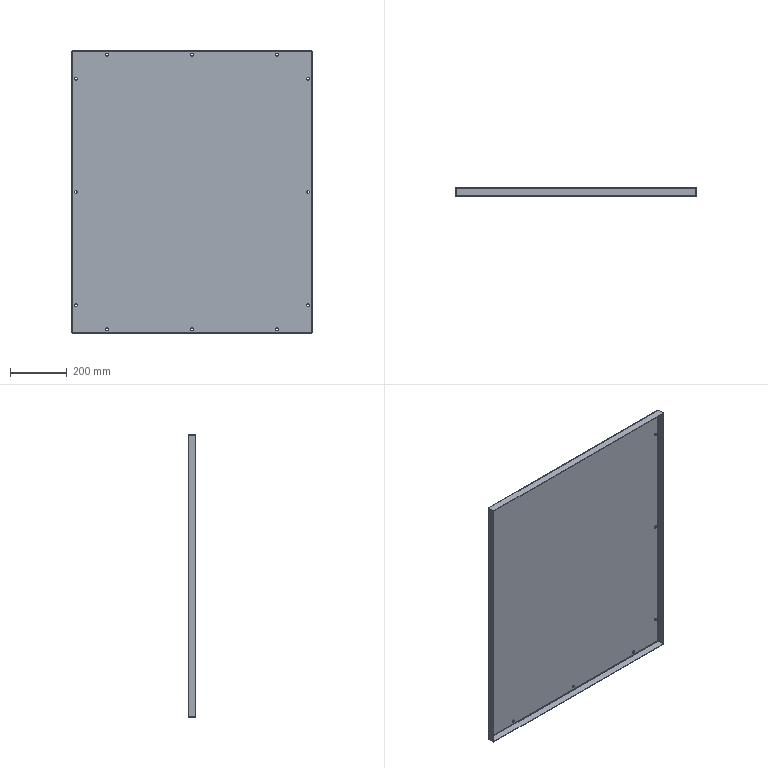Component | SolidWorks | 41TopPlateI-1 | 1 solid | 62 faces | volume 1883240 mm3 | cylinder 32 | plane 22 | spline 8 | commonest cylinder face diameters 10 x24 2 x4 6 x4